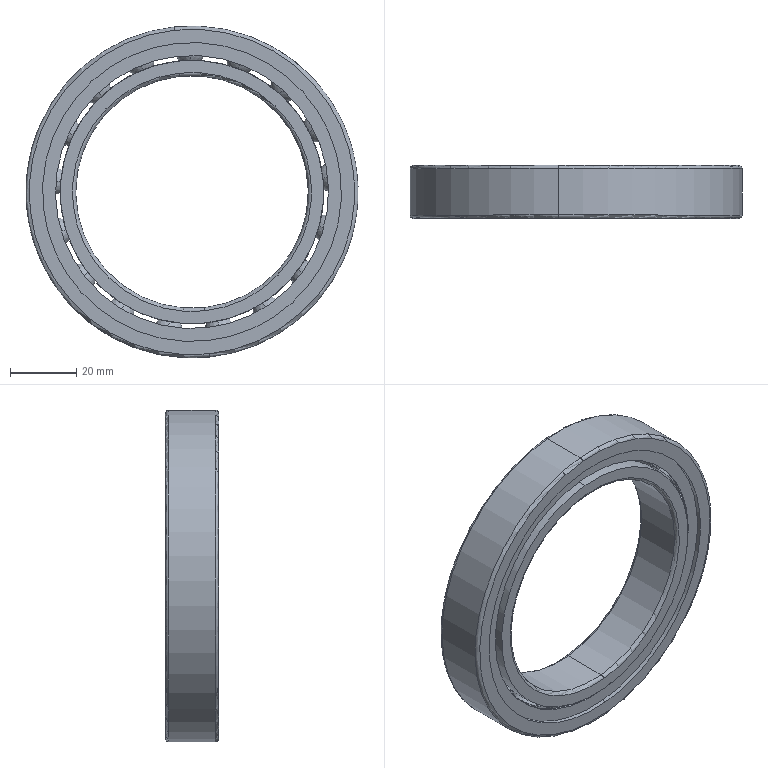Component | SolidWorks | LowerTensioningDeviceAssembly-1_GB_T276-94[DeepGrooveBallBearing61914-2Z]2-2 | 1 solid | 264 faces | volume 44871 mm3 | sphere 136 | torus 62 | plane 42 | cylinder 24 | commonest cylinder face diameters 90 x8 82.181 x4 79.3 x4 70 x2 100 x2 87.051 x2 82.249 x2